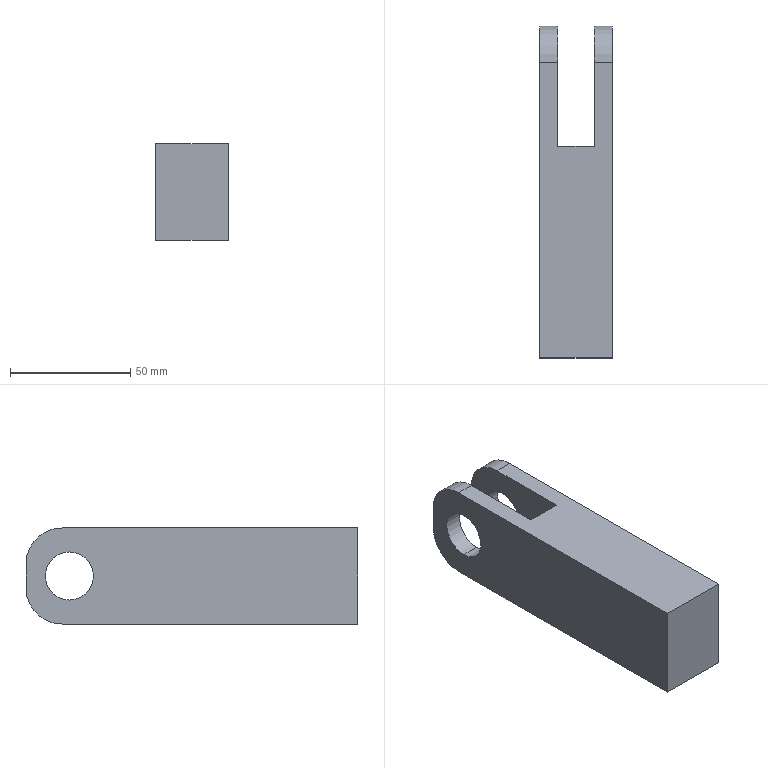Component | SolidWorks | HZ022-A001-D006-1 | 1 solid | 18 faces | box 30 x 138 x 40 mm | volume 129439 mm3 | plane 10 | cylinder 8 | commonest cylinder face diameters 20 x4 30 x4 | material AL6061
build123d program:
from build123d import *

# Parameters (mm, degrees)
SKETCH1_W           = 138
SKETCH1_H           = 40
BOSS_EXTRUDE1_DEPTH = 15
SKETCH2_R           = 10
CUT_EXTRUDE1_DEPTH  = 15
SKETCH3_W           = 50
SKETCH3_H           = 40
CUT_EXTRUDE2_DEPTH  = 7.5
FILLET1_R           = 15


with BuildPart() as part:
    # Sketch1 → Boss-Extrude1 (new, symmetric)
    with BuildSketch(Plane(origin=(0, 0, 0), x_dir=(1, 0, 0), z_dir=(0, 1, 0))):
        Rectangle(SKETCH1_W, SKETCH1_H)
    extrude(amount=BOSS_EXTRUDE1_DEPTH, both=True)

    # Sketch2 → Cut-Extrude1 (cut, symmetric)
    with BuildSketch(Plane(origin=(0, 0, 0), x_dir=(1, 0, 0), z_dir=(0, 1, 0))):
        with Locations(Location((-51, 0, 0), (0, 0, 270))):
            Circle(SKETCH2_R)
    extrude(amount=CUT_EXTRUDE1_DEPTH, both=True, mode=Mode.SUBTRACT)

    # Sketch3 → Cut-Extrude2 (cut, symmetric)
    with BuildSketch(Plane(origin=(0, 0, 0), x_dir=(1, 0, 0), z_dir=(0, 1, 0))):
        with Locations((-44, 0)):
            Rectangle(SKETCH3_W, SKETCH3_H)
    extrude(amount=CUT_EXTRUDE2_DEPTH, both=True, mode=Mode.SUBTRACT)

    # Fillet1
    fillet1_edges = [part.edges().sort_by_distance(p)[0] for p in [
        (-69, -11.25, 20),
        (-69, -11.25, -20),
        (-69, 11.25, 20),
        (-69, 11.25, -20),
    ]]
    fillet(fillet1_edges, radius=FILLET1_R)


solid = part.part

# Placed as in the assembly
solid = solid.moved(Location((-12.865, -2.602, 436), (0, 0, -90)))
STEP:
#1=COLOUR_RGB('',0.7922,0.8196,0.9333);
#2=FILL_AREA_STYLE_COLOUR('',#1);
#3=FILL_AREA_STYLE('',(#2));
#4=SURFACE_STYLE_FILL_AREA(#3);
#5=SURFACE_SIDE_STYLE('',(#4));
#6=SURFACE_STYLE_USAGE(.BOTH.,#5);
#7=PRESENTATION_STYLE_ASSIGNMENT((#6));
#8=CARTESIAN_POINT('',(-0.2112,1.905,17.559));
#9=VERTEX_POINT('',#8);
#10=CARTESIAN_POINT('',(-0.2112,1.905,16.772));
#11=VERTEX_POINT('',#10);
#12=CARTESIAN_POINT('',(-0.2112,1.905,17.165));
#13=DIRECTION('',(-1.,0.,0.));
#14=DIRECTION('',(0.,0.,1.));
#15=AXIS2_PLACEMENT_3D('',#12,#13,#14);
#16=CIRCLE('',#15,0.3937);
#17=EDGE_CURVE('',#9,#11,#16,.T.);
#18=ORIENTED_EDGE('',*,*,#17,.T.);
#19=CARTESIAN_POINT('',(0.08406,1.905,16.772));
#20=VERTEX_POINT('',#19);
#21=CARTESIAN_POINT('',(-1.097,1.905,16.772));
#22=DIRECTION('',(1.,0.,0.));
#23=VECTOR('',#22,39.37);
#24=LINE('',#21,#23);
#25=EDGE_CURVE('',#11,#20,#24,.T.);
#26=ORIENTED_EDGE('',*,*,#25,.T.);
#27=CARTESIAN_POINT('',(0.08406,1.905,17.559));
#28=VERTEX_POINT('',#27);
#29=CARTESIAN_POINT('',(0.08406,1.905,17.165));
#30=DIRECTION('',(1.,0.,0.));
#31=DIRECTION('',(0.,0.,1.));
#32=AXIS2_PLACEMENT_3D('',#29,#30,#31);
#33=CIRCLE('',#32,0.3937);
#34=EDGE_CURVE('',#20,#28,#33,.T.);
#35=ORIENTED_EDGE('',*,*,#34,.T.);
#36=CARTESIAN_POINT('',(-1.097,1.905,17.559));
#37=DIRECTION('',(1.,0.,0.));
#38=VECTOR('',#37,39.37);
#39=LINE('',#36,#38);
#40=EDGE_CURVE('',#9,#28,#39,.T.);
#41=ORIENTED_EDGE('',*,*,#40,.F.);
#42=EDGE_LOOP('',(#18,#26,#35,#41));
#43=FACE_OUTER_BOUND('',#42,.T.);
#44=CARTESIAN_POINT('',(-1.097,1.905,17.165));
#45=DIRECTION('',(1.,0.,0.));
#46=DIRECTION('',(0.,0.,1.));
#47=AXIS2_PLACEMENT_3D('',#44,#45,#46);
#48=CYLINDRICAL_SURFACE('',#47,0.3937);
#49=ADVANCED_FACE('',(#43),#48,.F.);
#50=CARTESIAN_POINT('',(-1.097,1.905,16.772));
#51=VERTEX_POINT('',#50);
#52=CARTESIAN_POINT('',(-1.097,1.905,17.559));
#53=VERTEX_POINT('',#52);
#54=CARTESIAN_POINT('',(-1.097,1.905,17.165));
#55=DIRECTION('',(1.,0.,0.));
#56=DIRECTION('',(0.,0.,1.));
#57=AXIS2_PLACEMENT_3D('',#54,#55,#56);
#58=CIRCLE('',#57,0.3937);
#59=EDGE_CURVE('',#51,#53,#58,.T.);
#60=ORIENTED_EDGE('',*,*,#59,.F.);
#61=CARTESIAN_POINT('',(-0.8018,1.905,16.772));
#62=VERTEX_POINT('',#61);
#63=CARTESIAN_POINT('',(-1.097,1.905,16.772));
#64=DIRECTION('',(1.,0.,0.));
#65=VECTOR('',#64,39.37);
#66=LINE('',#63,#65);
#67=EDGE_CURVE('',#51,#62,#66,.T.);
#68=ORIENTED_EDGE('',*,*,#67,.T.);
#69=CARTESIAN_POINT('',(-0.8018,1.905,17.559));
#70=VERTEX_POINT('',#69);
#71=CARTESIAN_POINT('',(-0.8018,1.905,17.165));
#72=DIRECTION('',(-1.,0.,0.));
#73=DIRECTION('',(0.,0.,1.));
#74=AXIS2_PLACEMENT_3D('',#71,#72,#73);
#75=CIRCLE('',#74,0.3937);
#76=EDGE_CURVE('',#70,#62,#75,.T.);
#77=ORIENTED_EDGE('',*,*,#76,.F.);
#78=CARTESIAN_POINT('',(-1.097,1.905,17.559));
#79=DIRECTION('',(1.,0.,0.));
#80=VECTOR('',#79,39.37);
#81=LINE('',#78,#80);
#82=EDGE_CURVE('',#53,#70,#81,.T.);
#83=ORIENTED_EDGE('',*,*,#82,.F.);
#84=EDGE_LOOP('',(#60,#68,#77,#83));
#85=FACE_OUTER_BOUND('',#84,.T.);
#86=CARTESIAN_POINT('',(-1.097,1.905,17.165));
#87=DIRECTION('',(1.,0.,0.));
#88=DIRECTION('',(0.,0.,1.));
#89=AXIS2_PLACEMENT_3D('',#86,#87,#88);
#90=CYLINDRICAL_SURFACE('',#89,0.3937);
#91=ADVANCED_FACE('',(#85),#90,.F.);
#92=CARTESIAN_POINT('',(-1.097,-2.819,16.378));
#93=VERTEX_POINT('',#92);
#94=CARTESIAN_POINT('',(-1.097,2.024,16.378));
#95=VERTEX_POINT('',#94);
#96=CARTESIAN_POINT('',(-1.097,2.614,16.378));
#97=DIRECTION('',(0.,1.,0.));
#98=VECTOR('',#97,39.37);
#99=LINE('',#96,#98);
#100=EDGE_CURVE('',#93,#95,#99,.T.);
#101=ORIENTED_EDGE('',*,*,#100,.T.);
#102=CARTESIAN_POINT('',(-0.8018,2.024,16.378));
#103=VERTEX_POINT('',#102);
#104=CARTESIAN_POINT('',(0.08406,2.024,16.378));
#105=DIRECTION('',(1.,0.,0.));
#106=VECTOR('',#105,39.37);
#107=LINE('',#104,#106);
#108=EDGE_CURVE('',#95,#103,#107,.T.);
#109=ORIENTED_EDGE('',*,*,#108,.T.);
#110=CARTESIAN_POINT('',(-0.8018,0.6456,16.378));
#111=VERTEX_POINT('',#110);
#112=CARTESIAN_POINT('',(-0.8018,2.614,16.378));
#113=DIRECTION('',(0.,1.,0.));
#114=VECTOR('',#113,39.37);
#115=LINE('',#112,#114);
#116=EDGE_CURVE('',#111,#103,#115,.T.);
#117=ORIENTED_EDGE('',*,*,#116,.F.);
#118=CARTESIAN_POINT('',(-0.2112,0.6456,16.378));
#119=VERTEX_POINT('',#118);
#120=CARTESIAN_POINT('',(-0.8018,0.6456,16.378));
#121=DIRECTION('',(1.,0.,0.));
#122=VECTOR('',#121,39.37);
#123=LINE('',#120,#122);
#124=EDGE_CURVE('',#111,#119,#123,.T.);
#125=ORIENTED_EDGE('',*,*,#124,.T.);
#126=CARTESIAN_POINT('',(-0.2112,2.024,16.378));
#127=VERTEX_POINT('',#126);
#128=CARTESIAN_POINT('',(-0.2112,2.614,16.378));
#129=DIRECTION('',(0.,1.,0.));
#130=VECTOR('',#129,39.37);
#131=LINE('',#128,#130);
#132=EDGE_CURVE('',#119,#127,#131,.T.);
#133=ORIENTED_EDGE('',*,*,#132,.T.);
#134=CARTESIAN_POINT('',(0.08406,2.024,16.378));
#135=VERTEX_POINT('',#134);
#136=CARTESIAN_POINT('',(0.08406,2.024,16.378));
#137=DIRECTION('',(1.,0.,0.));
#138=VECTOR('',#137,39.37);
#139=LINE('',#136,#138);
#140=EDGE_CURVE('',#127,#135,#139,.T.);
#141=ORIENTED_EDGE('',*,*,#140,.T.);
#142=CARTESIAN_POINT('',(0.08406,-2.819,16.378));
#143=VERTEX_POINT('',#142);
#144=CARTESIAN_POINT('',(0.08406,2.614,16.378));
#145=DIRECTION('',(0.,1.,0.));
#146=VECTOR('',#145,39.37);
#147=LINE('',#144,#146);
#148=EDGE_CURVE('',#143,#135,#147,.T.);
#149=ORIENTED_EDGE('',*,*,#148,.F.);
#150=CARTESIAN_POINT('',(0.08406,-2.819,16.378));
#151=DIRECTION('',(-1.,0.,0.));
#152=VECTOR('',#151,39.37);
#153=LINE('',#150,#152);
#154=EDGE_CURVE('',#143,#93,#153,.T.);
#155=ORIENTED_EDGE('',*,*,#154,.T.);
#156=EDGE_LOOP('',(#101,#109,#117,#125,#133,#141,#149,#155));
#157=FACE_OUTER_BOUND('',#156,.T.);
#158=CARTESIAN_POINT('',(0.08406,2.614,16.378));
#159=DIRECTION('',(0.,0.,1.));
#160=DIRECTION('',(0.,-1.,0.));
#161=AXIS2_PLACEMENT_3D('',#158,#159,#160);
#162=PLANE('',#161);
#163=ADVANCED_FACE('',(#157),#162,.F.);
#164=CARTESIAN_POINT('',(-0.8018,2.614,16.969));
#165=VERTEX_POINT('',#164);
#166=CARTESIAN_POINT('',(-0.8018,2.614,17.362));
#167=VERTEX_POINT('',#166);
#168=CARTESIAN_POINT('',(-0.8018,2.614,16.378));
#169=DIRECTION('',(0.,0.,1.));
#170=VECTOR('',#169,39.37);
#171=LINE('',#168,#170);
#172=EDGE_CURVE('',#165,#167,#171,.T.);
#173=ORIENTED_EDGE('',*,*,#172,.F.);
#174=CARTESIAN_POINT('',(-1.097,2.614,16.969));
#175=VERTEX_POINT('',#174);
#176=CARTESIAN_POINT('',(0.08406,2.614,16.969));
#177=DIRECTION('',(-1.,0.,0.));
#178=VECTOR('',#177,39.37);
#179=LINE('',#176,#178);
#180=EDGE_CURVE('',#165,#175,#179,.T.);
#181=ORIENTED_EDGE('',*,*,#180,.T.);
#182=CARTESIAN_POINT('',(-1.097,2.614,17.362));
#183=VERTEX_POINT('',#182);
#184=CARTESIAN_POINT('',(-1.097,2.614,16.378));
#185=DIRECTION('',(0.,0.,1.));
#186=VECTOR('',#185,39.37);
#187=LINE('',#184,#186);
#188=EDGE_CURVE('',#175,#183,#187,.T.);
#189=ORIENTED_EDGE('',*,*,#188,.T.);
#190=CARTESIAN_POINT('',(0.08406,2.614,17.362));
#191=DIRECTION('',(1.,0.,0.));
#192=VECTOR('',#191,39.37);
#193=LINE('',#190,#192);
#194=EDGE_CURVE('',#183,#167,#193,.T.);
#195=ORIENTED_EDGE('',*,*,#194,.T.);
#196=EDGE_LOOP('',(#173,#181,#189,#195));
#197=FACE_OUTER_BOUND('',#196,.T.);
#198=CARTESIAN_POINT('',(0.08406,2.614,16.378));
#199=DIRECTION('',(0.,-1.,0.));
#200=DIRECTION('',(0.,0.,-1.));
#201=AXIS2_PLACEMENT_3D('',#198,#199,#200);
#202=PLANE('',#201);
#203=ADVANCED_FACE('',(#197),#202,.F.);
#204=CARTESIAN_POINT('',(-0.8018,2.024,17.953));
#205=VERTEX_POINT('',#204);
#206=CARTESIAN_POINT('',(-0.8018,0.6456,17.953));
#207=VERTEX_POINT('',#206);
#208=CARTESIAN_POINT('',(-0.8018,2.614,17.953));
#209=DIRECTION('',(0.,-1.,0.));
#210=VECTOR('',#209,39.37);
#211=LINE('',#208,#210);
#212=EDGE_CURVE('',#205,#207,#211,.T.);
#213=ORIENTED_EDGE('',*,*,#212,.F.);
#214=CARTESIAN_POINT('',(-1.097,2.024,17.953));
#215=VERTEX_POINT('',#214);
#216=CARTESIAN_POINT('',(0.08406,2.024,17.953));
#217=DIRECTION('',(-1.,0.,0.));
#218=VECTOR('',#217,39.37);
#219=LINE('',#216,#218);
#220=EDGE_CURVE('',#205,#215,#219,.T.);
#221=ORIENTED_EDGE('',*,*,#220,.T.);
#222=CARTESIAN_POINT('',(-1.097,-2.819,17.953));
#223=VERTEX_POINT('',#222);
#224=CARTESIAN_POINT('',(-1.097,2.614,17.953));
#225=DIRECTION('',(0.,-1.,0.));
#226=VECTOR('',#225,39.37);
#227=LINE('',#224,#226);
#228=EDGE_CURVE('',#215,#223,#227,.T.);
#229=ORIENTED_EDGE('',*,*,#228,.T.);
#230=CARTESIAN_POINT('',(0.08406,-2.819,17.953));
#231=VERTEX_POINT('',#230);
#232=CARTESIAN_POINT('',(0.08406,-2.819,17.953));
#233=DIRECTION('',(-1.,0.,0.));
#234=VECTOR('',#233,39.37);
#235=LINE('',#232,#234);
#236=EDGE_CURVE('',#231,#223,#235,.T.);
#237=ORIENTED_EDGE('',*,*,#236,.F.);
#238=CARTESIAN_POINT('',(0.08406,2.024,17.953));
#239=VERTEX_POINT('',#238);
#240=CARTESIAN_POINT('',(0.08406,2.614,17.953));
#241=DIRECTION('',(0.,-1.,0.));
#242=VECTOR('',#241,39.37);
#243=LINE('',#240,#242);
#244=EDGE_CURVE('',#239,#231,#243,.T.);
#245=ORIENTED_EDGE('',*,*,#244,.F.);
#246=CARTESIAN_POINT('',(-0.2112,2.024,17.953));
#247=VERTEX_POINT('',#246);
#248=CARTESIAN_POINT('',(0.08406,2.024,17.953));
#249=DIRECTION('',(-1.,0.,0.));
#250=VECTOR('',#249,39.37);
#251=LINE('',#248,#250);
#252=EDGE_CURVE('',#239,#247,#251,.T.);
#253=ORIENTED_EDGE('',*,*,#252,.T.);
#254=CARTESIAN_POINT('',(-0.2112,0.6456,17.953));
#255=VERTEX_POINT('',#254);
#256=CARTESIAN_POINT('',(-0.2112,2.614,17.953));
#257=DIRECTION('',(0.,-1.,0.));
#258=VECTOR('',#257,39.37);
#259=LINE('',#256,#258);
#260=EDGE_CURVE('',#247,#255,#259,.T.);
#261=ORIENTED_EDGE('',*,*,#260,.T.);
#262=CARTESIAN_POINT('',(-0.8018,0.6456,17.953));
#263=DIRECTION('',(1.,0.,0.));
#264=VECTOR('',#263,39.37);
#265=LINE('',#262,#264);
#266=EDGE_CURVE('',#207,#255,#265,.T.);
#267=ORIENTED_EDGE('',*,*,#266,.F.);
#268=EDGE_LOOP('',(#213,#221,#229,#237,#245,#253,#261,#267));
#269=FACE_OUTER_BOUND('',#268,.T.);
#270=CARTESIAN_POINT('',(0.08406,2.614,17.953));
#271=DIRECTION('',(0.,0.,-1.));
#272=DIRECTION('',(0.,1.,0.));
#273=AXIS2_PLACEMENT_3D('',#270,#271,#272);
#274=PLANE('',#273);
#275=ADVANCED_FACE('',(#269),#274,.F.);
#276=ORIENTED_EDGE('',*,*,#67,.F.);
#277=CARTESIAN_POINT('',(-1.097,1.905,17.165));
#278=DIRECTION('',(1.,0.,0.));
#279=DIRECTION('',(0.,0.,1.));
#280=AXIS2_PLACEMENT_3D('',#277,#278,#279);
#281=CIRCLE('',#280,0.3937);
#282=EDGE_CURVE('',#53,#51,#281,.T.);
#283=ORIENTED_EDGE('',*,*,#282,.F.);
#284=ORIENTED_EDGE('',*,*,#82,.T.);
#285=CARTESIAN_POINT('',(-0.8018,1.905,17.165));
#286=DIRECTION('',(-1.,0.,0.));
#287=DIRECTION('',(0.,0.,1.));
#288=AXIS2_PLACEMENT_3D('',#285,#286,#287);
#289=CIRCLE('',#288,0.3937);
#290=EDGE_CURVE('',#62,#70,#289,.T.);
#291=ORIENTED_EDGE('',*,*,#290,.F.);
#292=EDGE_LOOP('',(#276,#283,#284,#291));
#293=FACE_OUTER_BOUND('',#292,.T.);
#294=CARTESIAN_POINT('',(-1.097,1.905,17.165));
#295=DIRECTION('',(1.,0.,0.));
#296=DIRECTION('',(0.,0.,1.));
#297=AXIS2_PLACEMENT_3D('',#294,#295,#296);
#298=CYLINDRICAL_SURFACE('',#297,0.3937);
#299=ADVANCED_FACE('',(#293),#298,.F.);
#300=CARTESIAN_POINT('',(-1.097,-2.819,16.378));
#301=DIRECTION('',(0.,0.,-1.));
#302=VECTOR('',#301,39.37);
#303=LINE('',#300,#302);
#304=EDGE_CURVE('',#223,#93,#303,.T.);
#305=ORIENTED_EDGE('',*,*,#304,.T.);
#306=ORIENTED_EDGE('',*,*,#154,.F.);
#307=CARTESIAN_POINT('',(0.08406,-2.819,16.378));
#308=DIRECTION('',(0.,0.,-1.));
#309=VECTOR('',#308,39.37);
#310=LINE('',#307,#309);
#311=EDGE_CURVE('',#231,#143,#310,.T.);
#312=ORIENTED_EDGE('',*,*,#311,.F.);
#313=ORIENTED_EDGE('',*,*,#236,.T.);
#314=EDGE_LOOP('',(#305,#306,#312,#313));
#315=FACE_OUTER_BOUND('',#314,.T.);
#316=CARTESIAN_POINT('',(0.08406,-2.819,16.378));
#317=DIRECTION('',(0.,1.,0.));
#318=DIRECTION('',(0.,0.,1.));
#319=AXIS2_PLACEMENT_3D('',#316,#317,#318);
#320=PLANE('',#319);
#321=ADVANCED_FACE('',(#315),#320,.F.);
#322=CARTESIAN_POINT('',(-0.2112,2.614,16.969));
#323=VERTEX_POINT('',#322);
#324=CARTESIAN_POINT('',(-0.2112,2.614,17.362));
#325=VERTEX_POINT('',#324);
#326=CARTESIAN_POINT('',(-0.2112,2.614,16.378));
#327=DIRECTION('',(0.,0.,1.));
#328=VECTOR('',#327,39.37);
#329=LINE('',#326,#328);
#330=EDGE_CURVE('',#323,#325,#329,.T.);
#331=ORIENTED_EDGE('',*,*,#330,.T.);
#332=CARTESIAN_POINT('',(0.08406,2.614,17.362));
#333=VERTEX_POINT('',#332);
#334=CARTESIAN_POINT('',(0.08406,2.614,17.362));
#335=DIRECTION('',(1.,0.,0.));
#336=VECTOR('',#335,39.37);
#337=LINE('',#334,#336);
#338=EDGE_CURVE('',#325,#333,#337,.T.);
#339=ORIENTED_EDGE('',*,*,#338,.T.);
#340=CARTESIAN_POINT('',(0.08406,2.614,16.969));
#341=VERTEX_POINT('',#340);
#342=CARTESIAN_POINT('',(0.08406,2.614,16.378));
#343=DIRECTION('',(0.,0.,1.));
#344=VECTOR('',#343,39.37);
#345=LINE('',#342,#344);
#346=EDGE_CURVE('',#341,#333,#345,.T.);
#347=ORIENTED_EDGE('',*,*,#346,.F.);
#348=CARTESIAN_POINT('',(0.08406,2.614,16.969));
#349=DIRECTION('',(-1.,0.,0.));
#350=VECTOR('',#349,39.37);
#351=LINE('',#348,#350);
#352=EDGE_CURVE('',#341,#323,#351,.T.);
#353=ORIENTED_EDGE('',*,*,#352,.T.);
#354=EDGE_LOOP('',(#331,#339,#347,#353));
#355=FACE_OUTER_BOUND('',#354,.T.);
#356=CARTESIAN_POINT('',(0.08406,2.614,16.378));
#357=DIRECTION('',(0.,-1.,0.));
#358=DIRECTION('',(0.,0.,-1.));
#359=AXIS2_PLACEMENT_3D('',#356,#357,#358);
#360=PLANE('',#359);
#361=ADVANCED_FACE('',(#355),#360,.F.);
#362=CARTESIAN_POINT('',(0.08406,1.905,17.165));
#363=DIRECTION('',(1.,0.,0.));
#364=DIRECTION('',(0.,0.,1.));
#365=AXIS2_PLACEMENT_3D('',#362,#363,#364);
#366=CIRCLE('',#365,0.3937);
#367=EDGE_CURVE('',#28,#20,#366,.T.);
#368=ORIENTED_EDGE('',*,*,#367,.F.);
#369=ORIENTED_EDGE('',*,*,#34,.F.);
#370=EDGE_LOOP('',(#368,#369));
#371=FACE_BOUND('',#370,.T.);
#372=ORIENTED_EDGE('',*,*,#346,.T.);
#373=CARTESIAN_POINT('',(0.08406,2.024,17.362));
#374=DIRECTION('',(1.,0.,0.));
#375=DIRECTION('',(0.,0.,1.));
#376=AXIS2_PLACEMENT_3D('',#373,#374,#375);
#377=CIRCLE('',#376,0.5906);
#378=EDGE_CURVE('',#333,#239,#377,.T.);
#379=ORIENTED_EDGE('',*,*,#378,.T.);
#380=ORIENTED_EDGE('',*,*,#244,.T.);
#381=ORIENTED_EDGE('',*,*,#311,.T.);
#382=ORIENTED_EDGE('',*,*,#148,.T.);
#383=CARTESIAN_POINT('',(0.08406,2.024,16.969));
#384=DIRECTION('',(1.,0.,0.));
#385=DIRECTION('',(0.,0.,1.));
#386=AXIS2_PLACEMENT_3D('',#383,#384,#385);
#387=CIRCLE('',#386,0.5906);
#388=EDGE_CURVE('',#135,#341,#387,.T.);
#389=ORIENTED_EDGE('',*,*,#388,.T.);
#390=EDGE_LOOP('',(#372,#379,#380,#381,#382,#389));
#391=FACE_OUTER_BOUND('',#390,.T.);
#392=CARTESIAN_POINT('',(0.08406,-0.1025,17.165));
#393=DIRECTION('',(1.,0.,0.));
#394=DIRECTION('',(0.,0.,1.));
#395=AXIS2_PLACEMENT_3D('',#392,#393,#394);
#396=PLANE('',#395);
#397=ADVANCED_FACE('',(#371,#391),#396,.T.);
#398=ORIENTED_EDGE('',*,*,#282,.T.);
#399=ORIENTED_EDGE('',*,*,#59,.T.);
#400=EDGE_LOOP('',(#398,#399));
#401=FACE_BOUND('',#400,.T.);
#402=ORIENTED_EDGE('',*,*,#188,.F.);
#403=CARTESIAN_POINT('',(-1.097,2.024,16.969));
#404=DIRECTION('',(-1.,0.,0.));
#405=DIRECTION('',(0.,0.,1.));
#406=AXIS2_PLACEMENT_3D('',#403,#404,#405);
#407=CIRCLE('',#406,0.5906);
#408=EDGE_CURVE('',#175,#95,#407,.T.);
#409=ORIENTED_EDGE('',*,*,#408,.T.);
#410=ORIENTED_EDGE('',*,*,#100,.F.);
#411=ORIENTED_EDGE('',*,*,#304,.F.);
#412=ORIENTED_EDGE('',*,*,#228,.F.);
#413=CARTESIAN_POINT('',(-1.097,2.024,17.362));
#414=DIRECTION('',(-1.,0.,0.));
#415=DIRECTION('',(0.,0.,1.));
#416=AXIS2_PLACEMENT_3D('',#413,#414,#415);
#417=CIRCLE('',#416,0.5906);
#418=EDGE_CURVE('',#215,#183,#417,.T.);
#419=ORIENTED_EDGE('',*,*,#418,.T.);
#420=EDGE_LOOP('',(#402,#409,#410,#411,#412,#419));
#421=FACE_OUTER_BOUND('',#420,.T.);
#422=CARTESIAN_POINT('',(-1.097,-0.1025,17.165));
#423=DIRECTION('',(1.,0.,0.));
#424=DIRECTION('',(0.,0.,1.));
#425=AXIS2_PLACEMENT_3D('',#422,#423,#424);
#426=PLANE('',#425);
#427=ADVANCED_FACE('',(#401,#421),#426,.F.);
#428=ORIENTED_EDGE('',*,*,#25,.F.);
#429=CARTESIAN_POINT('',(-0.2112,1.905,17.165));
#430=DIRECTION('',(-1.,0.,0.));
#431=DIRECTION('',(0.,0.,1.));
#432=AXIS2_PLACEMENT_3D('',#429,#430,#431);
#433=CIRCLE('',#432,0.3937);
#434=EDGE_CURVE('',#11,#9,#433,.T.);
#435=ORIENTED_EDGE('',*,*,#434,.T.);
#436=ORIENTED_EDGE('',*,*,#40,.T.);
#437=ORIENTED_EDGE('',*,*,#367,.T.);
#438=EDGE_LOOP('',(#428,#435,#436,#437));
#439=FACE_OUTER_BOUND('',#438,.T.);
#440=CARTESIAN_POINT('',(-1.097,1.905,17.165));
#441=DIRECTION('',(1.,0.,0.));
#442=DIRECTION('',(0.,0.,1.));
#443=AXIS2_PLACEMENT_3D('',#440,#441,#442);
#444=CYLINDRICAL_SURFACE('',#443,0.3937);
#445=ADVANCED_FACE('',(#439),#444,.F.);
#446=ORIENTED_EDGE('',*,*,#116,.T.);
#447=CARTESIAN_POINT('',(-0.8018,2.024,16.969));
#448=DIRECTION('',(1.,0.,0.));
#449=DIRECTION('',(0.,0.,1.));
#450=AXIS2_PLACEMENT_3D('',#447,#448,#449);
#451=CIRCLE('',#450,0.5906);
#452=EDGE_CURVE('',#103,#165,#451,.T.);
#453=ORIENTED_EDGE('',*,*,#452,.T.);
#454=ORIENTED_EDGE('',*,*,#172,.T.);
#455=CARTESIAN_POINT('',(-0.8018,2.024,17.362));
#456=DIRECTION('',(1.,0.,0.));
#457=DIRECTION('',(0.,0.,1.));
#458=AXIS2_PLACEMENT_3D('',#455,#456,#457);
#459=CIRCLE('',#458,0.5906);
#460=EDGE_CURVE('',#167,#205,#459,.T.);
#461=ORIENTED_EDGE('',*,*,#460,.T.);
#462=ORIENTED_EDGE('',*,*,#212,.T.);
#463=CARTESIAN_POINT('',(-0.8018,0.6456,16.378));
#464=DIRECTION('',(0.,0.,-1.));
#465=VECTOR('',#464,39.37);
#466=LINE('',#463,#465);
#467=EDGE_CURVE('',#207,#111,#466,.T.);
#468=ORIENTED_EDGE('',*,*,#467,.T.);
#469=EDGE_LOOP('',(#446,#453,#454,#461,#462,#468));
#470=FACE_OUTER_BOUND('',#469,.T.);
#471=ORIENTED_EDGE('',*,*,#76,.T.);
#472=ORIENTED_EDGE('',*,*,#290,.T.);
#473=EDGE_LOOP('',(#471,#472));
#474=FACE_BOUND('',#473,.T.);
#475=CARTESIAN_POINT('',(-0.8018,-0.1025,17.165));
#476=DIRECTION('',(1.,0.,0.));
#477=DIRECTION('',(0.,0.,1.));
#478=AXIS2_PLACEMENT_3D('',#475,#476,#477);
#479=PLANE('',#478);
#480=ADVANCED_FACE('',(#470,#474),#479,.T.);
#481=ORIENTED_EDGE('',*,*,#260,.F.);
#482=CARTESIAN_POINT('',(-0.2112,2.024,17.362));
#483=DIRECTION('',(-1.,0.,0.));
#484=DIRECTION('',(0.,0.,1.));
#485=AXIS2_PLACEMENT_3D('',#482,#483,#484);
#486=CIRCLE('',#485,0.5906);
#487=EDGE_CURVE('',#247,#325,#486,.T.);
#488=ORIENTED_EDGE('',*,*,#487,.T.);
#489=ORIENTED_EDGE('',*,*,#330,.F.);
#490=CARTESIAN_POINT('',(-0.2112,2.024,16.969));
#491=DIRECTION('',(-1.,0.,0.));
#492=DIRECTION('',(0.,0.,1.));
#493=AXIS2_PLACEMENT_3D('',#490,#491,#492);
#494=CIRCLE('',#493,0.5906);
#495=EDGE_CURVE('',#323,#127,#494,.T.);
#496=ORIENTED_EDGE('',*,*,#495,.T.);
#497=ORIENTED_EDGE('',*,*,#132,.F.);
#498=CARTESIAN_POINT('',(-0.2112,0.6456,16.378));
#499=DIRECTION('',(0.,0.,-1.));
#500=VECTOR('',#499,39.37);
#501=LINE('',#498,#500);
#502=EDGE_CURVE('',#255,#119,#501,.T.);
#503=ORIENTED_EDGE('',*,*,#502,.F.);
#504=EDGE_LOOP('',(#481,#488,#489,#496,#497,#503));
#505=FACE_OUTER_BOUND('',#504,.T.);
#506=ORIENTED_EDGE('',*,*,#17,.F.);
#507=ORIENTED_EDGE('',*,*,#434,.F.);
#508=EDGE_LOOP('',(#506,#507));
#509=FACE_BOUND('',#508,.T.);
#510=CARTESIAN_POINT('',(-0.2112,-0.1025,17.165));
#511=DIRECTION('',(1.,0.,0.));
#512=DIRECTION('',(0.,0.,1.));
#513=AXIS2_PLACEMENT_3D('',#510,#511,#512);
#514=PLANE('',#513);
#515=ADVANCED_FACE('',(#505,#509),#514,.F.);
#516=ORIENTED_EDGE('',*,*,#502,.T.);
#517=ORIENTED_EDGE('',*,*,#124,.F.);
#518=ORIENTED_EDGE('',*,*,#467,.F.);
#519=ORIENTED_EDGE('',*,*,#266,.T.);
#520=EDGE_LOOP('',(#516,#517,#518,#519));
#521=FACE_OUTER_BOUND('',#520,.T.);
#522=CARTESIAN_POINT('',(-0.8018,0.6456,16.378));
#523=DIRECTION('',(0.,-1.,-0.));
#524=DIRECTION('',(0.,0.,-1.));
#525=AXIS2_PLACEMENT_3D('',#522,#523,#524);
#526=PLANE('',#525);
#527=ADVANCED_FACE('',(#521),#526,.F.);
#528=ORIENTED_EDGE('',*,*,#452,.F.);
#529=ORIENTED_EDGE('',*,*,#108,.F.);
#530=ORIENTED_EDGE('',*,*,#408,.F.);
#531=ORIENTED_EDGE('',*,*,#180,.F.);
#532=EDGE_LOOP('',(#528,#529,#530,#531));
#533=FACE_OUTER_BOUND('',#532,.T.);
#534=CARTESIAN_POINT('',(0.08406,2.024,16.969));
#535=DIRECTION('',(-1.,0.,0.));
#536=DIRECTION('',(0.,0.,-1.));
#537=AXIS2_PLACEMENT_3D('',#534,#535,#536);
#538=CYLINDRICAL_SURFACE('',#537,0.5906);
#539=ADVANCED_FACE('',(#533),#538,.T.);
#540=ORIENTED_EDGE('',*,*,#460,.F.);
#541=ORIENTED_EDGE('',*,*,#194,.F.);
#542=ORIENTED_EDGE('',*,*,#418,.F.);
#543=ORIENTED_EDGE('',*,*,#220,.F.);
#544=EDGE_LOOP('',(#540,#541,#542,#543));
#545=FACE_OUTER_BOUND('',#544,.T.);
#546=CARTESIAN_POINT('',(0.08406,2.024,17.362));
#547=DIRECTION('',(-1.,0.,0.));
#548=DIRECTION('',(0.,0.,-1.));
#549=AXIS2_PLACEMENT_3D('',#546,#547,#548);
#550=CYLINDRICAL_SURFACE('',#549,0.5906);
#551=ADVANCED_FACE('',(#545),#550,.T.);
#552=ORIENTED_EDGE('',*,*,#378,.F.);
#553=ORIENTED_EDGE('',*,*,#338,.F.);
#554=ORIENTED_EDGE('',*,*,#487,.F.);
#555=ORIENTED_EDGE('',*,*,#252,.F.);
#556=EDGE_LOOP('',(#552,#553,#554,#555));
#557=FACE_OUTER_BOUND('',#556,.T.);
#558=CARTESIAN_POINT('',(0.08406,2.024,17.362));
#559=DIRECTION('',(-1.,0.,0.));
#560=DIRECTION('',(0.,0.,-1.));
#561=AXIS2_PLACEMENT_3D('',#558,#559,#560);
#562=CYLINDRICAL_SURFACE('',#561,0.5906);
#563=ADVANCED_FACE('',(#557),#562,.T.);
#564=ORIENTED_EDGE('',*,*,#388,.F.);
#565=ORIENTED_EDGE('',*,*,#140,.F.);
#566=ORIENTED_EDGE('',*,*,#495,.F.);
#567=ORIENTED_EDGE('',*,*,#352,.F.);
#568=EDGE_LOOP('',(#564,#565,#566,#567));
#569=FACE_OUTER_BOUND('',#568,.T.);
#570=CARTESIAN_POINT('',(0.08406,2.024,16.969));
#571=DIRECTION('',(-1.,0.,0.));
#572=DIRECTION('',(0.,0.,-1.));
#573=AXIS2_PLACEMENT_3D('',#570,#571,#572);
#574=CYLINDRICAL_SURFACE('',#573,0.5906);
#575=ADVANCED_FACE('',(#569),#574,.T.);
#576=CLOSED_SHELL('',(#49,#91,#163,#203,#275,#299,#321,#361,#397,#427,#445,#480,#515,#527,#539,#551,#563,#575));
#577=MANIFOLD_SOLID_BREP('',#576);
#578=STYLED_ITEM('',(#7),#577);
#579=PRESENTATION_LAYER_ASSIGNMENT('','',(#578));
#580=(LENGTH_UNIT()NAMED_UNIT(*)SI_UNIT($,.METRE.));
#581=LENGTH_MEASURE_WITH_UNIT(LENGTH_MEASURE(0.0254),#580);
#582=DIMENSIONAL_EXPONENTS(1.,0.,0.,0.,0.,0.,0.);
#583=(CONVERSION_BASED_UNIT('',#581)LENGTH_UNIT()NAMED_UNIT(#582));
#584=UNCERTAINTY_MEASURE_WITH_UNIT(LENGTH_MEASURE(0.00001),#583,'','');
#585=(NAMED_UNIT(*)PLANE_ANGLE_UNIT()SI_UNIT($,.RADIAN.));
#586=(NAMED_UNIT(*)SI_UNIT($,.STERADIAN.)SOLID_ANGLE_UNIT());
#587=(GEOMETRIC_REPRESENTATION_CONTEXT(3)GLOBAL_UNCERTAINTY_ASSIGNED_CONTEXT((#584))GLOBAL_UNIT_ASSIGNED_CONTEXT((#583,#585,#586))REPRESENTATION_CONTEXT('',''));
#588=MECHANICAL_DESIGN_GEOMETRIC_PRESENTATION_REPRESENTATION('',(#578),#587);
#589=CARTESIAN_POINT('',(0.,0.,0.));
#590=DIRECTION('',(0.,0.,1.));
#591=DIRECTION('',(1.,0.,0.));
#592=AXIS2_PLACEMENT_3D('',#589,#590,#591);
#593=(LENGTH_UNIT()NAMED_UNIT(*)SI_UNIT($,.METRE.));
#594=LENGTH_MEASURE_WITH_UNIT(LENGTH_MEASURE(0.0254),#593);
#595=DIMENSIONAL_EXPONENTS(1.,0.,0.,0.,0.,0.,0.);
#596=(CONVERSION_BASED_UNIT('',#594)LENGTH_UNIT()NAMED_UNIT(#595));
#597=UNCERTAINTY_MEASURE_WITH_UNIT(LENGTH_MEASURE(0.00001),#596,'','');
#598=(NAMED_UNIT(*)PLANE_ANGLE_UNIT()SI_UNIT($,.RADIAN.));
#599=(NAMED_UNIT(*)SI_UNIT($,.STERADIAN.)SOLID_ANGLE_UNIT());
#600=(GEOMETRIC_REPRESENTATION_CONTEXT(3)GLOBAL_UNCERTAINTY_ASSIGNED_CONTEXT((#597))GLOBAL_UNIT_ASSIGNED_CONTEXT((#596,#598,#599))REPRESENTATION_CONTEXT('',''));
#601=ADVANCED_BREP_SHAPE_REPRESENTATION('',(#577,#592),#600);